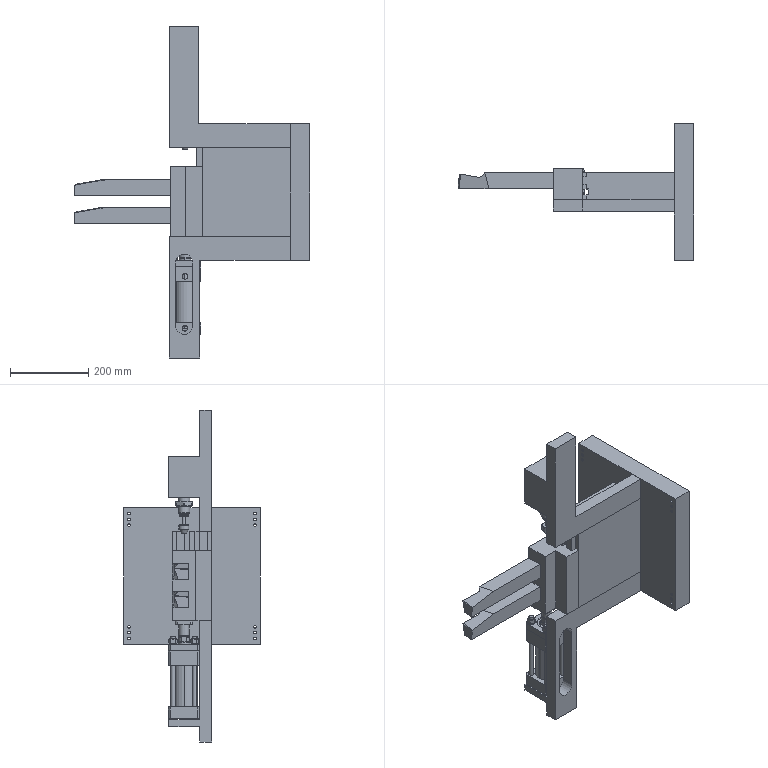Assembly | SolidWorks | mm | 32 component files | 34 solids | 685 faces | box 603.75 x 350 x 850 mm | volume 16732591 mm3 | plane 278 | cylinder 264 | cone 93 | torus 36 | spline 14 | commonest cylinder face diameters 12 x28 6.793 x24 14 x24 12.9 x24 19.1 x24 50 x18 47.059 x14 30 x12
Bill of materials:
FrontEndCap | 1 |  | Square block with chamfered vertical corners, four corner through-holes, a central stepped (multi-diameter) bore, a cross hole in one side face, and a short grooved cylindrical spigot on the opposite face.
Gland | 1 |  | Flat square plate with chamfered corners, four corner through-holes and a large central through-bore with a small edge step or chamfer.
GuideSleeve | 1 |  | Flanged cylindrical bushing: short tube with a thin radial flange at one end and a stepped through-bore.
GB_FASTENER_NUT_SNAB1XY M12X1.5-N | 4 |  | Hexagonal prism with a central through-bore and chamfered corners on both end faces; hex-nut-like shape.
GB_FASTENER_NUT_SNAB1XY  B M18X1.5-N | 1 |  | Hexagonal prism with a central through-bore and chamfered corners on both ends; hex-nut-like shape, shown rotated about its axis in the end view.
Piston | 1 |  | Spool-like cylindrical part with four radial flanges (two end flanges with chamfered outer edges, two intermediate) separated by recessed cylindrical sections, with a central through-bore that has a step near one end.
PistonRod | 1 |  | Long stepped round shaft with a square, rounded-corner flange plate at one end carrying four small holes; the shaft has a short neck, a collar/step region, a long main diameter, and two progressively smaller stepped diameters at the far end.
RearEndCap | 1 |  | Square block with chamfered vertical corners, four corner through-holes, a raised grooved cylindrical boss on the top face with a central bore, and a cross hole in one side face; underside shows a shallow circular recess with a small off-centre feature.
GB_FASTENER_WASHER_SW 12 | 8 |  | Flat circular ring with a rectangular cross-section, cut through at one point by a single slanted radial gap; split-washer-like shape.
GB_FASTENER_WASHER_SW 18 | 1 |  | Flat circular ring with a rectangular cross-section and a single slanted radial split; split-washer-like shape.
SteelBarrel | 1 |  | Plain thin-walled cylindrical tube with open ends.
TieRod | 4 |  | Slender solid cylindrical rod with flat ends.
Fixture | 1 |  | Straight prismatic extrusion with a stepped profile: a wide portion and a narrower stem portion, with three rectangular notches cut along one long side of the profile.
HydraulicBufferACA1007-1AIRTAC | 1 |  | Cylindrical body carrying two hex nuts, with a small stepped end boss bearing a notch at one end and a thin rod at the other end terminating in a cylindrical head with a conical tip.
LatheTool | 2 |  | Rectangular-section straight bar with one end having a sloped and curved (scooped) top surface.
MirrorPlate | 1 |  | L-shaped bar of rectangular section with a rectangular block projecting sideways from the vertical leg.
Part8 | 1 |  | T-section block: a large flat square plate with a solid rectangular web standing out at right angles from the middle of one face. The web is not as tall as the plate, and its free end has stepped tabs and notches. The plate has small through-holes in four groups of three, one group near each corner.
PlateLeft | 1 |  | Bracket: a rectangular upright with a long rounded-end (obround) through-slot, a long straight rectangular arm sticking out sideways from the top of the upright, and a thin square flange plate near the bottom of the upright with four round through-holes.
Mates:
1. coincident | Part8-1 face at (-130.557, 55.832, -117.351) dir (0, 1, 0) | Fixture-2 face at (-136.557, 55.832, 62.649) dir (0, 1, 0)
2. coincident | Part8-1 face at (-136.557, 25.332, 172.649) dir (-1, 0, 0) | Fixture-2 face at (-136.557, 55.832, 62.649) dir (1, 0, 0)
3. coincident | Part8-1 face at (89.443, 180.832, -177.351) dir (0, 0, -1) | PlateLeft-1 face at (-220.557, -13.588, -177.351) dir (0, 0, -1)
4. coincident | Part8-1 face at (-130.557, -44.168, -117.351) dir (0, -1, 0) | PlateLeft-1 face at (-220.557, -44.168, -177.351) dir (0, -1, 0)
5. coincident | LatheTool-1 face at (-169.83, 14.482, -83.461) dir (0, 0, -1) | Fixture-2 face at (-216.557, 25.832, -83.461) dir (0, 0, 1)
6. coincident | LatheTool-1 face at (-169.83, 55.832, -42.111) dir (0, 1, 0) | Fixture-2 face at (-136.557, 55.832, 62.649) dir (0, 1, 0)
7. coincident | LatheTool-1 face at (-169.83, 35.157, -62.786) dir (1, 0, 0) | Fixture-2 face at (-169.83, 25.832, -83.461) dir (-1, 0, 0)
8. coincident | LatheTool-2 face at (-169.83, 14.482, 28.759) dir (0, 0, 1) | Fixture-2 face at (-136.557, 25.832, 28.759) dir (0, 0, -1)
9. coincident | LatheTool-2 face at (-169.83, 55.832, 28.759) dir (0, 1, 0) | Fixture-2 face at (-136.557, 55.832, 62.649) dir (0, 1, 0)
10. coincident | LatheTool-2 face at (-169.83, 35.157, 8.084) dir (1, 0, 0) | Fixture-2 face at (-169.83, 25.832, -117.351) dir (-1, 0, 0)
11. coincident | Part8-1 face at (89.443, -11.952, -528.526) dir (-1, 0, 0) | PlateLeft-1 face at (89.443, 0, 0) dir (1, 0, 0)
12. coincident | PlateLeft-1 face at (-220.557, -13.588, -177.351) dir (0, 1, 0) | Cylinder-1/FrontEndCap-1 face at (-140.557, -13.588, -194.351) dir (0, -1, 0)
13. coincident | PlateLeft-1 face at (-220.557, 0, 0) dir (-1, 0, 0) | Cylinder-1/FrontEndCap-1 face at (-220.557, 66.412, -194.351) dir (-1, 0, 0)
14. parallel | MirrorPlate-2 face at (89.443, 0, 422.649) dir (0, 0, 1) | HydraulicBufferACA1007-1AIRTAC-1 face at (-176.4, 28.812, 293.649) dir (0, 0, 1)
15. parallel | MirrorPlate-2 face at (-220.557, -13.588, 172.649) dir (0, 1, 0) | HydraulicBufferACA1007-1AIRTAC-1 face at (-192.681, 5.412, 197.649) dir (0, -1, 0)
16. concentric | Cylinder-1/PistonRod-2 face at (-180.557, 26.412, -72.093) dir (0, 0, 1) r 13 | HydraulicBufferACA1007-1AIRTAC-1 face at (-180.557, 26.412, 218.649) dir (0, 0, 1) r 15
17. coincident | MirrorPlate-2 face at (-145.557, 66.412, 197.649) dir (0, 0, -1) | HydraulicBufferACA1007-1AIRTAC-1 face at (-165.795, 34.935, 197.649) dir (0, 0, -1)
18. coincident | Fixture-2 face at (-136.557, 55.832, -117.351) dir (0, 0, -1) | Cylinder-1/PistonRod-2 face at (-180.557, 26.412, -117.351) dir (0, 0, 1)
19. parallel | Fixture-2 face at (-136.557, 55.832, 62.649) dir (0, 1, 0) | Cylinder-1/PistonRod-2 face at (-202.043, 48.358, -127.351) dir (0, 1, 0)
20. distance | Cylinder-1/RearEndCap-1 face at (-220.557, 66.412, -367.351) dir (0, 0, -1) | PlateLeft-1 face at (89.443, 0, -427.351) dir (0, 0, -1)
21. coincident | Gland-1 face at (30.07, 48.299, 30.558) dir (1, 0, 0) | FrontEndCap-1 face at (30.07, -31.701, 30.558) dir (-1, 0, 0)
22. concentric | Gland-1 face at (13.07, 8.299, -9.442) dir (1, 0, 0) r 25 | FrontEndCap-1 face at (48.07, 8.299, -9.442) dir (1, 0, 0) r 17.5
23. coincident | Gland-1 face at (13.07, 48.299, -49.442) dir (0, 0, -1) | FrontEndCap-1 face at (30.07, -31.701, -49.442) dir (0, 0, -1)
24. concentric | GuideSleeve-1 face at (56.795, 8.299, -9.442) dir (1, 0, 0) r 15 | Gland-1 face at (13.07, 8.299, -9.442) dir (1, 0, 0) r 25
25. coincident | GuideSleeve-1 face at (13.07, 1.807, 6.27) dir (-1, 0, 0) | Gland-1 face at (13.07, 48.299, 30.558) dir (-1, 0, 0)
26. coincident | Piston-1 face at (163.07, 18.299, -9.442) dir (1, 0, 0) | RearEndCap-1 face at (163.07, 48.299, 30.558) dir (-1, 0, 0)
27. concentric | Piston-1 face at (83.863, 8.299, -9.442) dir (-1, 0, 0) r 10 | RearEndCap-1 face at (193.07, 8.299, -9.442) dir (-1, 0, 0) r 17.5
28. coincident | FrontEndCap-1 face at (30.07, -31.701, -49.442) dir (0, 0, -1) | RearEndCap-1 face at (203.07, 48.299, -49.442) dir (0, 0, -1)
29. coincident | FrontEndCap-1 face at (68.07, 8.299, -34.442) dir (1, 0, 0) | SteelBarrel-1 face at (68.07, 8.299, -9.442) dir (-1, 0, 0)
30. concentric | FrontEndCap-1 face at (78.07, 36.299, -37.442) dir (-1, 0, 0) r 7 | TieRod-4 face at (-5.83, 36.299, -37.442) dir (1, 0, 0) r 6
31. concentric | FrontEndCap-1 face at (78.07, 36.299, 18.558) dir (-1, 0, 0) r 7 | TieRod-3 face at (-5.83, 36.299, 18.558) dir (1, 0, 0) r 6
32. concentric | FrontEndCap-1 face at (78.07, -19.701, 18.558) dir (-1, 0, 0) r 7 | TieRod-2 face at (-5.83, -19.701, 18.558) dir (1, 0, 0) r 6
33. concentric | FrontEndCap-1 face at (78.07, -19.701, -37.442) dir (-1, 0, 0) r 7 | TieRod-1 face at (-5.83, -19.701, -37.442) dir (1, 0, 0) r 6
34. coincident | TieRod-3 face at (-5.83, 36.299, 18.558) dir (-1, 0, 0) | TieRod-4 face at (-5.83, 36.299, -37.442) dir (-1, 0, 0)
35. coincident | TieRod-2 face at (-5.83, -19.701, 18.558) dir (-1, 0, 0) | TieRod-3 face at (-5.83, 36.299, 18.558) dir (-1, 0, 0)
36. coincident | TieRod-1 face at (-5.83, -19.701, -37.442) dir (-1, 0, 0) | TieRod-2 face at (-5.83, -19.701, 18.558) dir (-1, 0, 0)
37. concentric | TieRod-2 face at (-5.83, -19.701, 18.558) dir (1, 0, 0) r 6 | hex nuts 1-fine pitch-grades ab gb-6 face at (9.97, -19.701, 18.558) dir (-1, 0, 0) r 6
38. concentric | TieRod-3 face at (-5.83, 36.299, 18.558) dir (1, 0, 0) r 6 | hex nuts 1-fine pitch-grades ab gb-5 face at (9.97, 36.299, 18.558) dir (-1, 0, 0) r 6
39. concentric | TieRod-1 face at (-5.83, -19.701, -37.442) dir (1, 0, 0) r 6 | hex nuts 1-fine pitch-grades ab gb-4 face at (9.97, -19.701, -37.442) dir (-1, 0, 0) r 6
40. concentric | TieRod-4 face at (-5.83, 36.299, -37.442) dir (1, 0, 0) r 6 | hex nuts 1-fine pitch-grades ab gb-2 face at (9.97, 36.299, -37.442) dir (-1, 0, 0) r 6
41. coincident | hex nuts 1-fine pitch-grades ab gb-5 face at (-0.8298, 27.299, 2.97) dir (-1, 0, 0) | hex nuts 1-fine pitch-grades ab gb-6 face at (-0.8298, -28.701, 2.97) dir (-1, 0, 0)
42. coincident | hex nuts 1-fine pitch-grades ab gb-2 face at (-0.8298, 27.299, -53.03) dir (-1, 0, 0) | hex nuts 1-fine pitch-grades ab gb-5 face at (-0.8298, 27.299, 2.97) dir (-1, 0, 0)
43. coincident | hex nuts 1-fine pitch-grades ab gb-4 face at (-0.8298, -28.701, -53.03) dir (-1, 0, 0) | hex nuts 1-fine pitch-grades ab gb-6 face at (-0.8298, -28.701, 2.97) dir (-1, 0, 0)
44. concentric | hex nuts 1-fine pitch-grades ab gb-4 face at (9.97, -19.701, -37.442) dir (-1, 0, 0) r 6 | spring lock washers--normal type gb-4 face at (9.97, -19.701, -37.442) dir (1, 0, 0) r 6.45
45. coincident | hex nuts 1-fine pitch-grades ab gb-4 face at (9.97, -28.701, -53.03) dir (1, 0, 0) | spring lock washers--normal type gb-4 face at (9.97, -19.701, -37.442) dir (-1, 0, 0)
46. concentric | hex nuts 1-fine pitch-grades ab gb-6 face at (9.97, -19.701, 18.558) dir (-1, 0, 0) r 6 | spring lock washers--normal type gb-3 face at (9.97, -19.701, 18.558) dir (1, 0, 0) r 6.45
47. coincident | hex nuts 1-fine pitch-grades ab gb-6 face at (9.97, -28.701, 2.97) dir (1, 0, 0) | spring lock washers--normal type gb-3 face at (9.97, -19.701, 18.558) dir (-1, 0, 0)
48. concentric | hex nuts 1-fine pitch-grades ab gb-5 face at (9.97, 36.299, 18.558) dir (-1, 0, 0) r 6 | spring lock washers--normal type gb-2 face at (9.97, 36.299, 18.558) dir (1, 0, 0) r 6.45
49. coincident | hex nuts 1-fine pitch-grades ab gb-5 face at (9.97, 27.299, 2.97) dir (1, 0, 0) | spring lock washers--normal type gb-2 face at (9.97, 36.299, 18.558) dir (-1, 0, 0)
50. concentric | hex nuts 1-fine pitch-grades ab gb-2 face at (9.97, 36.299, -37.442) dir (-1, 0, 0) r 6 | spring lock washers--normal type gb-1 face at (9.97, 36.299, -37.442) dir (1, 0, 0) r 6.45
51. coincident | hex nuts 1-fine pitch-grades ab gb-2 face at (9.97, 27.299, -53.03) dir (1, 0, 0) | spring lock washers--normal type gb-1 face at (9.97, 36.299, -37.442) dir (-1, 0, 0)
52. coincident | Gland-1 face at (13.07, 48.299, 30.558) dir (-1, 0, 0) | spring lock washers--normal type gb-1 face at (13.07, 36.299, -37.442) dir (1, 0, 0)
53. coincident | RearEndCap-1 face at (173.07, 8.299, -34.442) dir (-1, 0, 0) | SteelBarrel-1 face at (173.07, 8.299, -9.442) dir (1, 0, 0)
54. distance | TieRod-4 face at (-5.83, 36.299, -37.442) dir (-1, 0, 0) | hex nuts 1-fine pitch-grades ab gb-2 face at (-0.8298, 27.299, -53.03) dir (-1, 0, 0)
55. concentric | TieRod-4 face at (-5.83, 36.299, -37.442) dir (1, 0, 0) r 6 | spring lock washers--normal type gb-6 face at (206.17, 36.299, -37.442) dir (-1, 0, 0) r 6.45
56. concentric | TieRod-3 face at (-5.83, 36.299, 18.558) dir (1, 0, 0) r 6 | spring lock washers--normal type gb-9 face at (206.17, 36.299, 18.558) dir (-1, 0, 0) r 6.45
57. concentric | TieRod-2 face at (-5.83, -19.701, 18.558) dir (1, 0, 0) r 6 | spring lock washers--normal type gb-5 face at (206.17, -19.701, 18.558) dir (-1, 0, 0) r 6.45
58. coincident | RearEndCap-1 face at (203.07, 48.299, 30.558) dir (1, 0, 0) | spring lock washers--normal type gb-6 face at (203.07, 36.299, -37.442) dir (-1, 0, 0)
59. coincident | spring lock washers--normal type gb-6 face at (206.17, 36.299, -37.442) dir (1, 0, 0) | spring lock washers--normal type gb-9 face at (206.17, 36.299, 18.558) dir (1, 0, 0)
60. coincident | RearEndCap-1 face at (203.07, 48.299, 30.558) dir (1, 0, 0) | spring lock washers--normal type gb-5 face at (203.07, -19.701, 18.558) dir (-1, 0, 0)
61. concentric | TieRod-1 face at (-5.83, -19.701, -37.442) dir (1, 0, 0) r 6 | spring lock washers--normal type gb-10 face at (206.17, -19.701, -37.442) dir (-1, 0, 0) r 6.45
62. coincident | RearEndCap-1 face at (203.07, 48.299, 30.558) dir (1, 0, 0) | spring lock washers--normal type gb-10 face at (203.07, -19.701, -37.442) dir (-1, 0, 0)
63. coincident | hex nuts 1-fine pitch-grades ab gb-9 face at (167.57, -2.658, 1.646) dir (-1, 0, 0) | spring lock washers--normal type gb-11 face at (167.57, 8.299, -9.442) dir (1, 0, 0)
64. concentric | hex nuts 1-fine pitch-grades ab gb-9 face at (167.57, 8.299, -9.442) dir (1, 0, 0) r 9 | spring lock washers--normal type gb-11 face at (163.07, 8.299, -9.442) dir (1, 0, 0) r 9.52
65. coincident | Piston-1 face at (163.07, 18.299, -9.442) dir (1, 0, 0) | spring lock washers--normal type gb-11 face at (163.07, 8.299, -9.442) dir (-1, 0, 0)
66. concentric | GuideSleeve-1 face at (56.795, 8.299, -9.442) dir (1, 0, 0) r 15 | PistonRod-2 face at (-92.188, 8.299, -9.442) dir (-1, 0, 0) r 15
67. concentric | RearEndCap-1 face at (203.07, 8.299, -9.442) dir (1, 0, 0) r 25 | SteelBarrel-1 face at (68.07, 8.299, -9.442) dir (1, 0, 0) r 25
68. concentric | Piston-1 face at (83.863, 8.299, -9.442) dir (-1, 0, 0) r 25 | spring lock washers--normal type gb-11 face at (163.07, 8.299, -9.442) dir (1, 0, 0) r 9.52
69. coincident | Piston-1 face at (128.07, 32.799, -9.442) dir (-1, 0, 0) | PistonRod-2 face at (128.07, 23.299, -9.442) dir (1, 0, 0)